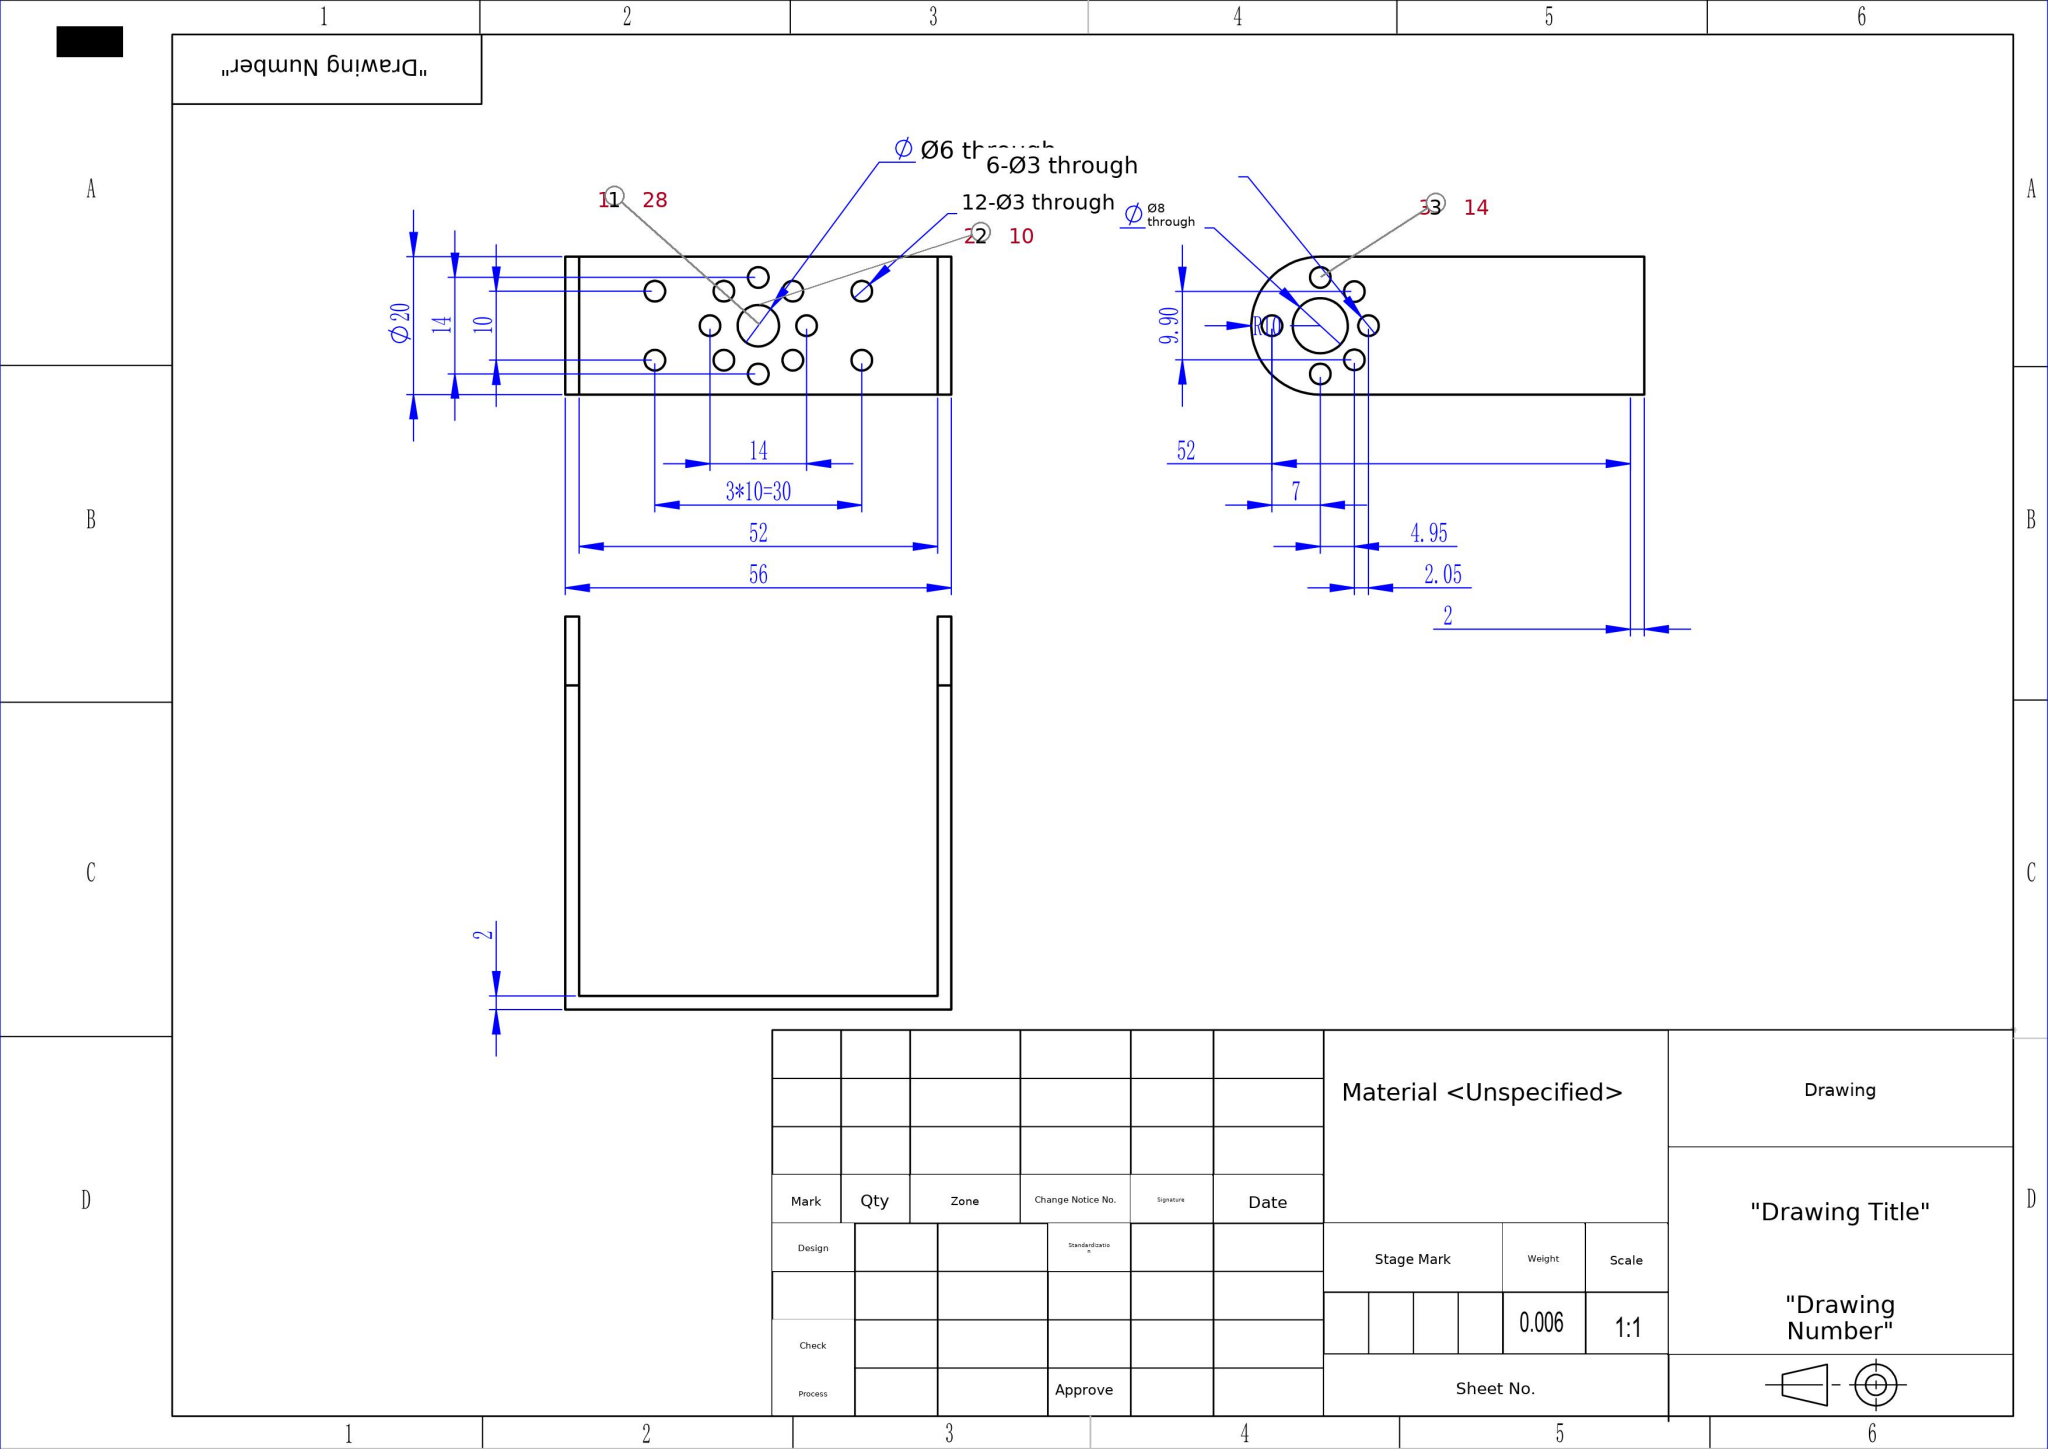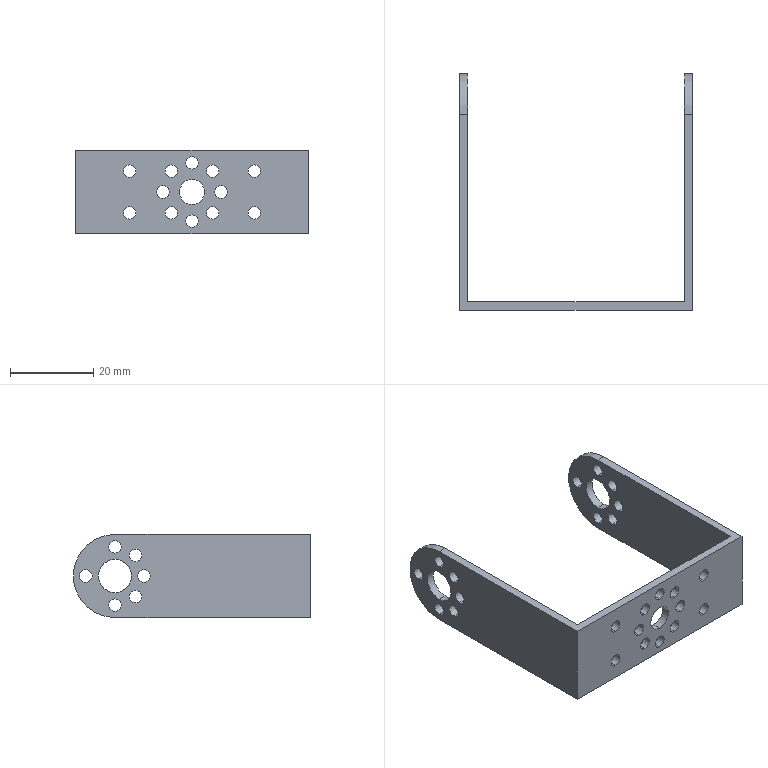Part | SolidWorks | mm | 1 solid | 64 faces | box 56 x 57 x 20 mm | volume 5871 mm3 | cylinder 56 | plane 8 | commonest cylinder face diameters 3 x48 8 x4 6 x2 20 x2
build123d program:
from build123d import *

# Parameters (mm, degrees)
SKETCH1_W           = 56
SKETCH1_H           = 20
BOSS_EXTRUDE1_DEPTH = 2
CUT_EXTRUDE1_REACH  = 61.498
SKETCH2_R           = 3
SKETCH2_R_2         = 1.5
BOSS_EXTRUDE2_DEPTH = 2
CUT_EXTRUDE2_REACH  = 84.371
SKETCH4_R           = 4
SKETCH4_R_2         = 1.5


with BuildPart() as part:
    # Sketch1 → Boss-Extrude1 (new body)
    with BuildSketch(Plane(origin=(0, 0, 0), x_dir=(1, 0, 0), z_dir=(0, 1, 0))):
        with Locations((28, 10)):
            Rectangle(SKETCH1_W, SKETCH1_H)
    extrude(amount=BOSS_EXTRUDE1_DEPTH)

    # Sketch2 → Cut-Extrude1 (cut, up to next)
    with BuildSketch(Plane(origin=(0, 2, 0), x_dir=(1, 0, 0), z_dir=(0, 1, 0)), mode=Mode.PRIVATE) as cut_extrude1_sk1:
        with Locations(Location((28, 10, 0), (0, 0, 270))):
            Circle(SKETCH2_R)
    cut_extrude1_tool1 = extrude(cut_extrude1_sk1.sketch, amount=-CUT_EXTRUDE1_REACH, mode=Mode.PRIVATE) & part.part
    # Sketch2 → Cut-Extrude1 (cut, up to next)
    with BuildSketch(Plane(origin=(0, 2, 0), x_dir=(1, 0, 0), z_dir=(0, 1, 0)), mode=Mode.PRIVATE) as cut_extrude1_sk2:
        with Locations(Location((28, 17, 0), (0, 0, 270))):
            Circle(SKETCH2_R_2)
    cut_extrude1_tool2 = extrude(cut_extrude1_sk2.sketch, amount=-CUT_EXTRUDE1_REACH, mode=Mode.PRIVATE) & part.part
    # Sketch2 → Cut-Extrude1 (cut, up to next)
    with BuildSketch(Plane(origin=(0, 2, 0), x_dir=(1, 0, 0), z_dir=(0, 1, 0)), mode=Mode.PRIVATE) as cut_extrude1_sk3:
        with Locations(Location((33, 5, 0), (0, 0, 270))):
            Circle(SKETCH2_R_2)
    cut_extrude1_tool3 = extrude(cut_extrude1_sk3.sketch, amount=-CUT_EXTRUDE1_REACH, mode=Mode.PRIVATE) & part.part
    # Sketch2 → Cut-Extrude1 (cut, up to next)
    with BuildSketch(Plane(origin=(0, 2, 0), x_dir=(1, 0, 0), z_dir=(0, 1, 0)), mode=Mode.PRIVATE) as cut_extrude1_sk4:
        with Locations(Location((23, 5, 0), (0, 0, 270))):
            Circle(SKETCH2_R_2)
    cut_extrude1_tool4 = extrude(cut_extrude1_sk4.sketch, amount=-CUT_EXTRUDE1_REACH, mode=Mode.PRIVATE) & part.part
    # Sketch2 → Cut-Extrude1 (cut, up to next)
    with BuildSketch(Plane(origin=(0, 2, 0), x_dir=(1, 0, 0), z_dir=(0, 1, 0)), mode=Mode.PRIVATE) as cut_extrude1_sk5:
        with Locations(Location((23, 15, 0), (0, 0, 270))):
            Circle(SKETCH2_R_2)
    cut_extrude1_tool5 = extrude(cut_extrude1_sk5.sketch, amount=-CUT_EXTRUDE1_REACH, mode=Mode.PRIVATE) & part.part
    # Sketch2 → Cut-Extrude1 (cut, up to next)
    with BuildSketch(Plane(origin=(0, 2, 0), x_dir=(1, 0, 0), z_dir=(0, 1, 0)), mode=Mode.PRIVATE) as cut_extrude1_sk6:
        with Locations(Location((33, 15, 0), (0, 0, 270))):
            Circle(SKETCH2_R_2)
    cut_extrude1_tool6 = extrude(cut_extrude1_sk6.sketch, amount=-CUT_EXTRUDE1_REACH, mode=Mode.PRIVATE) & part.part
    # Sketch2 → Cut-Extrude1 (cut, up to next)
    with BuildSketch(Plane(origin=(0, 2, 0), x_dir=(1, 0, 0), z_dir=(0, 1, 0)), mode=Mode.PRIVATE) as cut_extrude1_sk7:
        with Locations(Location((21, 10, 0), (0, 0, 270))):
            Circle(SKETCH2_R_2)
    cut_extrude1_tool7 = extrude(cut_extrude1_sk7.sketch, amount=-CUT_EXTRUDE1_REACH, mode=Mode.PRIVATE) & part.part
    # Sketch2 → Cut-Extrude1 (cut, up to next)
    with BuildSketch(Plane(origin=(0, 2, 0), x_dir=(1, 0, 0), z_dir=(0, 1, 0)), mode=Mode.PRIVATE) as cut_extrude1_sk8:
        with Locations(Location((13, 15, 0), (0, 0, 270))):
            Circle(SKETCH2_R_2)
    cut_extrude1_tool8 = extrude(cut_extrude1_sk8.sketch, amount=-CUT_EXTRUDE1_REACH, mode=Mode.PRIVATE) & part.part
    # Sketch2 → Cut-Extrude1 (cut, up to next)
    with BuildSketch(Plane(origin=(0, 2, 0), x_dir=(1, 0, 0), z_dir=(0, 1, 0)), mode=Mode.PRIVATE) as cut_extrude1_sk9:
        with Locations(Location((13, 5, 0), (0, 0, 90))):
            Circle(SKETCH2_R_2)
    cut_extrude1_tool9 = extrude(cut_extrude1_sk9.sketch, amount=-CUT_EXTRUDE1_REACH, mode=Mode.PRIVATE) & part.part
    # Sketch2 → Cut-Extrude1 (cut, up to next)
    with BuildSketch(Plane(origin=(0, 2, 0), x_dir=(1, 0, 0), z_dir=(0, 1, 0)), mode=Mode.PRIVATE) as cut_extrude1_sk10:
        with Locations(Location((43, 5, 0), (0, 0, 270))):
            Circle(SKETCH2_R_2)
    cut_extrude1_tool10 = extrude(cut_extrude1_sk10.sketch, amount=-CUT_EXTRUDE1_REACH, mode=Mode.PRIVATE) & part.part
    # Sketch2 → Cut-Extrude1 (cut, up to next)
    with BuildSketch(Plane(origin=(0, 2, 0), x_dir=(1, 0, 0), z_dir=(0, 1, 0)), mode=Mode.PRIVATE) as cut_extrude1_sk11:
        with Locations(Location((43, 15, 0), (0, 0, 90))):
            Circle(SKETCH2_R_2)
    cut_extrude1_tool11 = extrude(cut_extrude1_sk11.sketch, amount=-CUT_EXTRUDE1_REACH, mode=Mode.PRIVATE) & part.part
    # Sketch2 → Cut-Extrude1 (cut, up to next)
    with BuildSketch(Plane(origin=(0, 2, 0), x_dir=(1, 0, 0), z_dir=(0, 1, 0)), mode=Mode.PRIVATE) as cut_extrude1_sk12:
        with Locations(Location((35, 10, 0), (0, 0, 270))):
            Circle(SKETCH2_R_2)
    cut_extrude1_tool12 = extrude(cut_extrude1_sk12.sketch, amount=-CUT_EXTRUDE1_REACH, mode=Mode.PRIVATE) & part.part
    # Sketch2 → Cut-Extrude1 (cut, up to next)
    with BuildSketch(Plane(origin=(0, 2, 0), x_dir=(1, 0, 0), z_dir=(0, 1, 0)), mode=Mode.PRIVATE) as cut_extrude1_sk13:
        with Locations(Location((28, 3, 0), (0, 0, 270))):
            Circle(SKETCH2_R_2)
    cut_extrude1_tool13 = extrude(cut_extrude1_sk13.sketch, amount=-CUT_EXTRUDE1_REACH, mode=Mode.PRIVATE) & part.part
    add(cut_extrude1_tool1.solids().sort_by_distance((28, 2, -10))[0], mode=Mode.SUBTRACT)
    add(cut_extrude1_tool2.solids().sort_by_distance((28, 2, -17))[0], mode=Mode.SUBTRACT)
    add(cut_extrude1_tool3.solids().sort_by_distance((33, 2, -5))[0], mode=Mode.SUBTRACT)
    add(cut_extrude1_tool4.solids().sort_by_distance((23, 2, -5))[0], mode=Mode.SUBTRACT)
    add(cut_extrude1_tool5.solids().sort_by_distance((23, 2, -15))[0], mode=Mode.SUBTRACT)
    add(cut_extrude1_tool6.solids().sort_by_distance((33, 2, -15))[0], mode=Mode.SUBTRACT)
    add(cut_extrude1_tool7.solids().sort_by_distance((21, 2, -10))[0], mode=Mode.SUBTRACT)
    add(cut_extrude1_tool8.solids().sort_by_distance((13, 2, -15))[0], mode=Mode.SUBTRACT)
    add(cut_extrude1_tool9.solids().sort_by_distance((13, 2, -5))[0], mode=Mode.SUBTRACT)
    add(cut_extrude1_tool10.solids().sort_by_distance((43, 2, -5))[0], mode=Mode.SUBTRACT)
    add(cut_extrude1_tool11.solids().sort_by_distance((43, 2, -15))[0], mode=Mode.SUBTRACT)
    add(cut_extrude1_tool12.solids().sort_by_distance((35, 2, -10))[0], mode=Mode.SUBTRACT)
    add(cut_extrude1_tool13.solids().sort_by_distance((28, 2, -3))[0], mode=Mode.SUBTRACT)

    # Sketch3 → Boss-Extrude2 (add)
    with BuildSketch(Plane.ZY):
        with BuildLine():
            Line((-20, 2), (0, 2))
            Line((0, 2), (0, 47))
            ThreePointArc((0, 47), (-10, 57), (-20, 47))
            Line((-20, 47), (-20, 2))
        make_face()
    boss_extrude2 = extrude(amount=-BOSS_EXTRUDE2_DEPTH)

    # Sketch4 → Cut-Extrude2 (cut, up to next)
    with BuildSketch(Plane.ZY, mode=Mode.PRIVATE) as cut_extrude2_sk1:
        with Locations((-10, 47)):
            Circle(SKETCH4_R)
    cut_extrude2_tool1 = extrude(cut_extrude2_sk1.sketch, amount=-CUT_EXTRUDE2_REACH, mode=Mode.PRIVATE) & part.part
    # Sketch4 → Cut-Extrude2 (cut, up to next)
    with BuildSketch(Plane.ZY, mode=Mode.PRIVATE) as cut_extrude2_sk2:
        with Locations((-10, 54)):
            Circle(SKETCH4_R_2)
    cut_extrude2_tool2 = extrude(cut_extrude2_sk2.sketch, amount=-CUT_EXTRUDE2_REACH, mode=Mode.PRIVATE) & part.part
    # Sketch4 → Cut-Extrude2 (cut, up to next)
    with BuildSketch(Plane.ZY, mode=Mode.PRIVATE) as cut_extrude2_sk3:
        with Locations((-3, 47)):
            Circle(SKETCH4_R_2)
    cut_extrude2_tool3 = extrude(cut_extrude2_sk3.sketch, amount=-CUT_EXTRUDE2_REACH, mode=Mode.PRIVATE) & part.part
    # Sketch4 → Cut-Extrude2 (cut, up to next)
    with BuildSketch(Plane.ZY, mode=Mode.PRIVATE) as cut_extrude2_sk4:
        with Locations((-5.05, 42.05)):
            Circle(SKETCH4_R_2)
    cut_extrude2_tool4 = extrude(cut_extrude2_sk4.sketch, amount=-CUT_EXTRUDE2_REACH, mode=Mode.PRIVATE) & part.part
    # Sketch4 → Cut-Extrude2 (cut, up to next)
    with BuildSketch(Plane.ZY, mode=Mode.PRIVATE) as cut_extrude2_sk5:
        with Locations((-10, 40)):
            Circle(SKETCH4_R_2)
    cut_extrude2_tool5 = extrude(cut_extrude2_sk5.sketch, amount=-CUT_EXTRUDE2_REACH, mode=Mode.PRIVATE) & part.part
    # Sketch4 → Cut-Extrude2 (cut, up to next)
    with BuildSketch(Plane.ZY, mode=Mode.PRIVATE) as cut_extrude2_sk6:
        with Locations((-14.95, 42.05)):
            Circle(SKETCH4_R_2)
    cut_extrude2_tool6 = extrude(cut_extrude2_sk6.sketch, amount=-CUT_EXTRUDE2_REACH, mode=Mode.PRIVATE) & part.part
    # Sketch4 → Cut-Extrude2 (cut, up to next)
    with BuildSketch(Plane.ZY, mode=Mode.PRIVATE) as cut_extrude2_sk7:
        with Locations((-17, 47)):
            Circle(SKETCH4_R_2)
    cut_extrude2_tool7 = extrude(cut_extrude2_sk7.sketch, amount=-CUT_EXTRUDE2_REACH, mode=Mode.PRIVATE) & part.part
    cut_extrude2_1 = cut_extrude2_tool1.solids().sort_by_distance((0, 47, -10))[0]
    add(cut_extrude2_1, mode=Mode.SUBTRACT)
    cut_extrude2_2 = cut_extrude2_tool2.solids().sort_by_distance((0, 54, -10))[0]
    add(cut_extrude2_2, mode=Mode.SUBTRACT)
    cut_extrude2_3 = cut_extrude2_tool3.solids().sort_by_distance((0, 47, -3))[0]
    add(cut_extrude2_3, mode=Mode.SUBTRACT)
    cut_extrude2_4 = cut_extrude2_tool4.solids().sort_by_distance((0, 42.05, -5.05))[0]
    add(cut_extrude2_4, mode=Mode.SUBTRACT)
    cut_extrude2_5 = cut_extrude2_tool5.solids().sort_by_distance((0, 40, -10))[0]
    add(cut_extrude2_5, mode=Mode.SUBTRACT)
    cut_extrude2_6 = cut_extrude2_tool6.solids().sort_by_distance((0, 42.05, -14.95))[0]
    add(cut_extrude2_6, mode=Mode.SUBTRACT)
    cut_extrude2_7 = cut_extrude2_tool7.solids().sort_by_distance((0, 47, -17))[0]
    add(cut_extrude2_7, mode=Mode.SUBTRACT)
    cut_extrude2 = cut_extrude2_1 + cut_extrude2_2 + cut_extrude2_3 + cut_extrude2_4 + cut_extrude2_5 + cut_extrude2_6 + cut_extrude2_7  # Cut-Extrude2 as one shape, for the pattern or mirror that repeats it

    # Mirror1: Boss-Extrude2, Cut-Extrude2 across plane
    add(boss_extrude2.mirror(Plane.ZY.offset(-28)))
    add(cut_extrude2.mirror(Plane.ZY.offset(-28)), mode=Mode.SUBTRACT)


solid = part.part